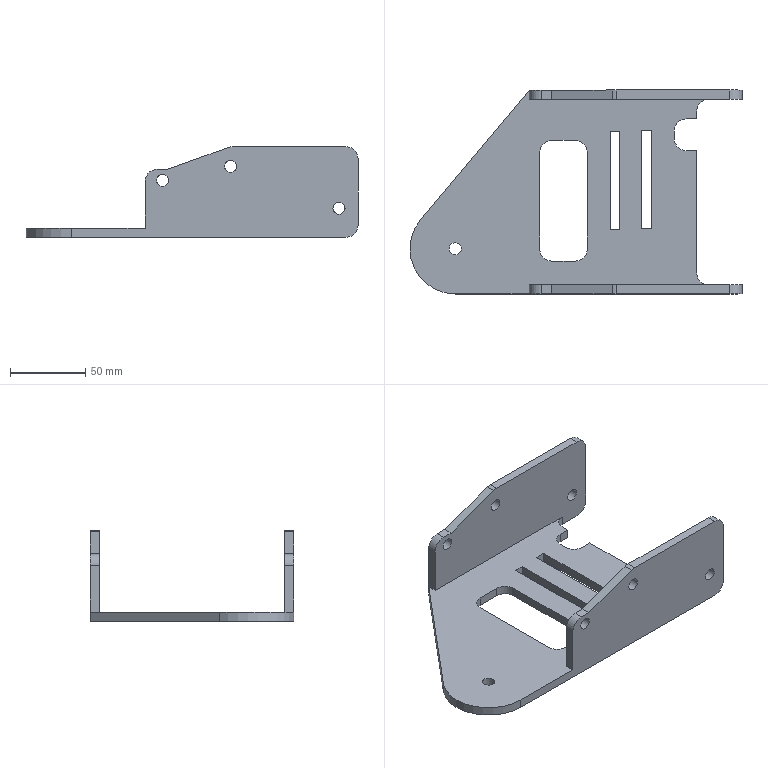Component | NX | BODY | 1 solid | 58 faces | volume 193536 mm3 | plane 34 | cylinder 24 | commonest cylinder face diameters 16 x16 8 x7 60 x1